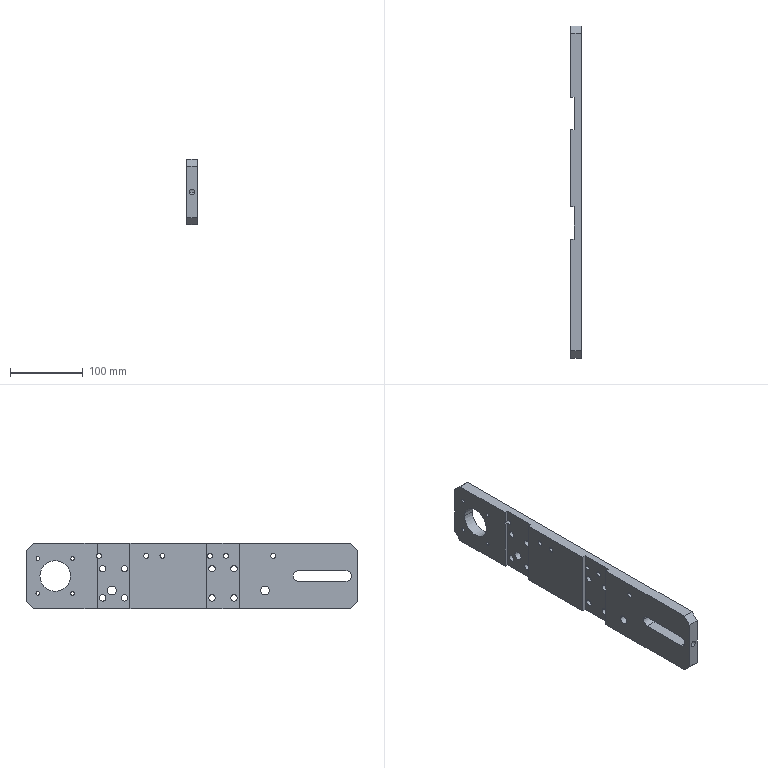Component | SolidWorks | LowerSideBeltXG-XG1-1_LowerRollerMountingPlateAXG-XG1-1 | 1 solid | 92 faces | box 15 x 455 x 90 mm | volume 516183 mm3 | cylinder 51 | plane 21 | cone 20 | commonest cylinder face diameters 6.8 x16 9 x16 5 x8 12 x4 15 x3 8.2 x2 42 x2
build123d program:
from build123d import *

# Parameters (mm, degrees)
SKETCH1_W                                           = 455
SKETCH1_H                                           = 90
BOSS_EXTRUDE1_DEPTH                                 = 7.5
M12_TAPPED_HOLE1_D                                  = 12
TAPERED_COUNTERSUNK_HOLE_FOR_M8_HEXAGON_D           = 9
TAPERED_COUNTERSUNK_HOLE_FOR_M8_HEXAGON_CSINK_D     = 17.92
TAPERED_COUNTERSUNK_HOLE_FOR_M8_HEXAGON_CSINK_ANGLE = 90
M8_TAPPED_HOLE1_D                                   = 6.8
SKETCH11_R                                          = 21
CUT_EXTRUDE1_DEPTH                                  = 15
M6_TAPPED_HOLE4_D                                   = 5
CIRPATTERN1_COUNT                                   = 4
CUT_EXTRUDE2_DEPTH                                  = 15
CHAMFER1_SIZE                                       = 10
CUT_EXTRUDE3_REACH                                  = 459.281
CUT_EXTRUDE3_END_RADIUS                             = 7.5
SKETCH23_R                                          = 4.1
CUT_EXTRUDE4_DEPTH                                  = 233.392
M8_TAPPED_HOLE2_D                                   = 6.8
M8_TAPPED_HOLE2_DEPTH                               = 15.75
M8_TAPPED_HOLE2_TIP                                 = 2.043
SKETCH27_W                                          = 45
SKETCH27_H                                          = 21.131
SKETCH27_H_2                                        = 19.025
CUT_EXTRUDE5_DEPTH                                  = 245.77


with BuildPart() as part:
    # Sketch1 → Boss-Extrude1 (new, symmetric)
    with BuildSketch(Plane.XY):
        Rectangle(SKETCH1_W, SKETCH1_H)
    extrude(amount=BOSS_EXTRUDE1_DEPTH, both=True)

    # M12 Tapped Hole1 (through all)
    with Locations(Plane(origin=(0, 0, -7.5), x_dir=(1, 0, 0), z_dir=(0, 0, -1))):
        with Locations((110, 20), (-100, 20)):
            Hole(M12_TAPPED_HOLE1_D / 2)

    # Tapered Countersunk Hole for M8 Hexagon (through all)
    with Locations(Plane.XY.offset(7.5)):
        with Locations((122.5, 10), (122.5, -30), (92.5, 10), (92.5, -30), (-27.5, -30), (-57.5, -30), (-57.5, 10), (-27.5, 10)):
            CounterSinkHole(TAPERED_COUNTERSUNK_HOLE_FOR_M8_HEXAGON_D / 2, TAPERED_COUNTERSUNK_HOLE_FOR_M8_HEXAGON_CSINK_D / 2, counter_sink_angle=TAPERED_COUNTERSUNK_HOLE_FOR_M8_HEXAGON_CSINK_ANGLE)

    # M8 Tapped Hole1 (through all)
    with Locations(Plane.XY.offset(7.5)):
        with Locations((127.5, 27.5), (62.5, 27.5), (40.5, 27.5), (-24.5, 27.5), (-46.5, 27.5), (-111.5, 27.5)):
            Hole(M8_TAPPED_HOLE1_D / 2)

    # Sketch11 → Cut-Extrude1 (cut)
    with BuildSketch(Plane.XY.offset(7.5)):
        with Locations((187.5, 0)):
            Circle(SKETCH11_R)
    extrude(amount=-CUT_EXTRUDE1_DEPTH, mode=Mode.SUBTRACT)

    # M6 Tapped Hole4 (through all)
    with Locations(Plane.XY.offset(7.5)):
        with Locations((163.635, 23.865)):
            m6_tapped_hole4 = Hole(M6_TAPPED_HOLE4_D / 2)

    # CirPattern1: M6 Tapped Hole4 ×4 about axis
    cirpattern1_axis = Axis((187.5, 0, 0), (0, 0, 1))
    for i in range(1, CIRPATTERN1_COUNT):
        add(m6_tapped_hole4.rotate(cirpattern1_axis, i * 360 / CIRPATTERN1_COUNT), mode=Mode.SUBTRACT)

    # Sketch14 → Cut-Extrude2 (cut)
    with BuildSketch(Plane.XY.offset(7.5)):
        with BuildLine():
            Line((-211, 7.5), (-151, 7.5))
            ThreePointArc((-151, 7.5), (-143.5, 0), (-151, -7.5))
            Line((-151, -7.5), (-211, -7.5))
            ThreePointArc((-211, -7.5), (-218.5, 0), (-211, 7.5))
        make_face()
    extrude(amount=-CUT_EXTRUDE2_DEPTH, mode=Mode.SUBTRACT)

    # Chamfer1
    chamfer1_edges = [part.edges().sort_by_distance(p)[0] for p in [
        (227.5, -45, 0),
        (-227.5, -45, 0),
        (-227.5, 45, 0),
        (227.5, 45, 0),
    ]]
    chamfer(chamfer1_edges, length=CHAMFER1_SIZE)

    # Cut-Extrude3: up to this cylinder (the profile starts outside it)
    cut_extrude3_end = Plane(origin=(-211, 0, 0), z_dir=(0, 0, 1)) * Cylinder(CUT_EXTRUDE3_END_RADIUS, 934.562, mode=Mode.PRIVATE)
    # Sketch23 → Cut-Extrude3 (cut, up to the surface)
    with BuildSketch(Plane.ZY.offset(227.5), mode=Mode.PRIVATE) as cut_extrude3_sk1:
        Circle(SKETCH23_R)
    cut_extrude3_tool1 = extrude(cut_extrude3_sk1.sketch, amount=-CUT_EXTRUDE3_REACH, mode=Mode.PRIVATE) - cut_extrude3_end
    add(cut_extrude3_tool1.solids().sort_by_distance((-227.5, 0, 0))[0], mode=Mode.SUBTRACT)

    # Sketch24 → Cut-Extrude4 (cut, through all)
    with BuildSketch(Plane.XY.offset(7.5)):
        with BuildLine():
            Line((-151, 7.5), (-146, 7.5))
            ThreePointArc((-146, 7.5), (-138.5, 0), (-146, -7.5))
            Line((-146, -7.5), (-151, -7.5))
            Line((-151, -7.5), (-151, 7.5))
        make_face()
    extrude(amount=-CUT_EXTRUDE4_DEPTH, mode=Mode.SUBTRACT)

    # M8 Tapped Hole2
    with Locations(Plane.XZ.offset(45)):
        with Locations((17.5, 0), (47.5, 0)):
            Hole(M8_TAPPED_HOLE2_D / 2, depth=M8_TAPPED_HOLE2_DEPTH)
            with Locations((0, 0, -(M8_TAPPED_HOLE2_DEPTH + M8_TAPPED_HOLE2_TIP / 2))):  # 118° drill point
                Cone(0, M8_TAPPED_HOLE2_D / 2, M8_TAPPED_HOLE2_TIP, mode=Mode.SUBTRACT)

    # Sketch27 → Cut-Extrude5 (cut, through all)
    with BuildSketch(Plane(origin=(0, 45, 0), x_dir=(1, 0, 0), z_dir=(0, 1, 0))):
        with Locations((-42.5, 13.066)):
            Rectangle(SKETCH27_W, SKETCH27_H)
        with Locations((107.5, 12.013)):
            Rectangle(SKETCH27_W, SKETCH27_H_2)
    extrude(amount=-CUT_EXTRUDE5_DEPTH, mode=Mode.SUBTRACT)


solid = part.part

# Placed as in the assembly
solid = solid.moved(Location((-323.72, 437.5, 114), (90, 90, 0)))